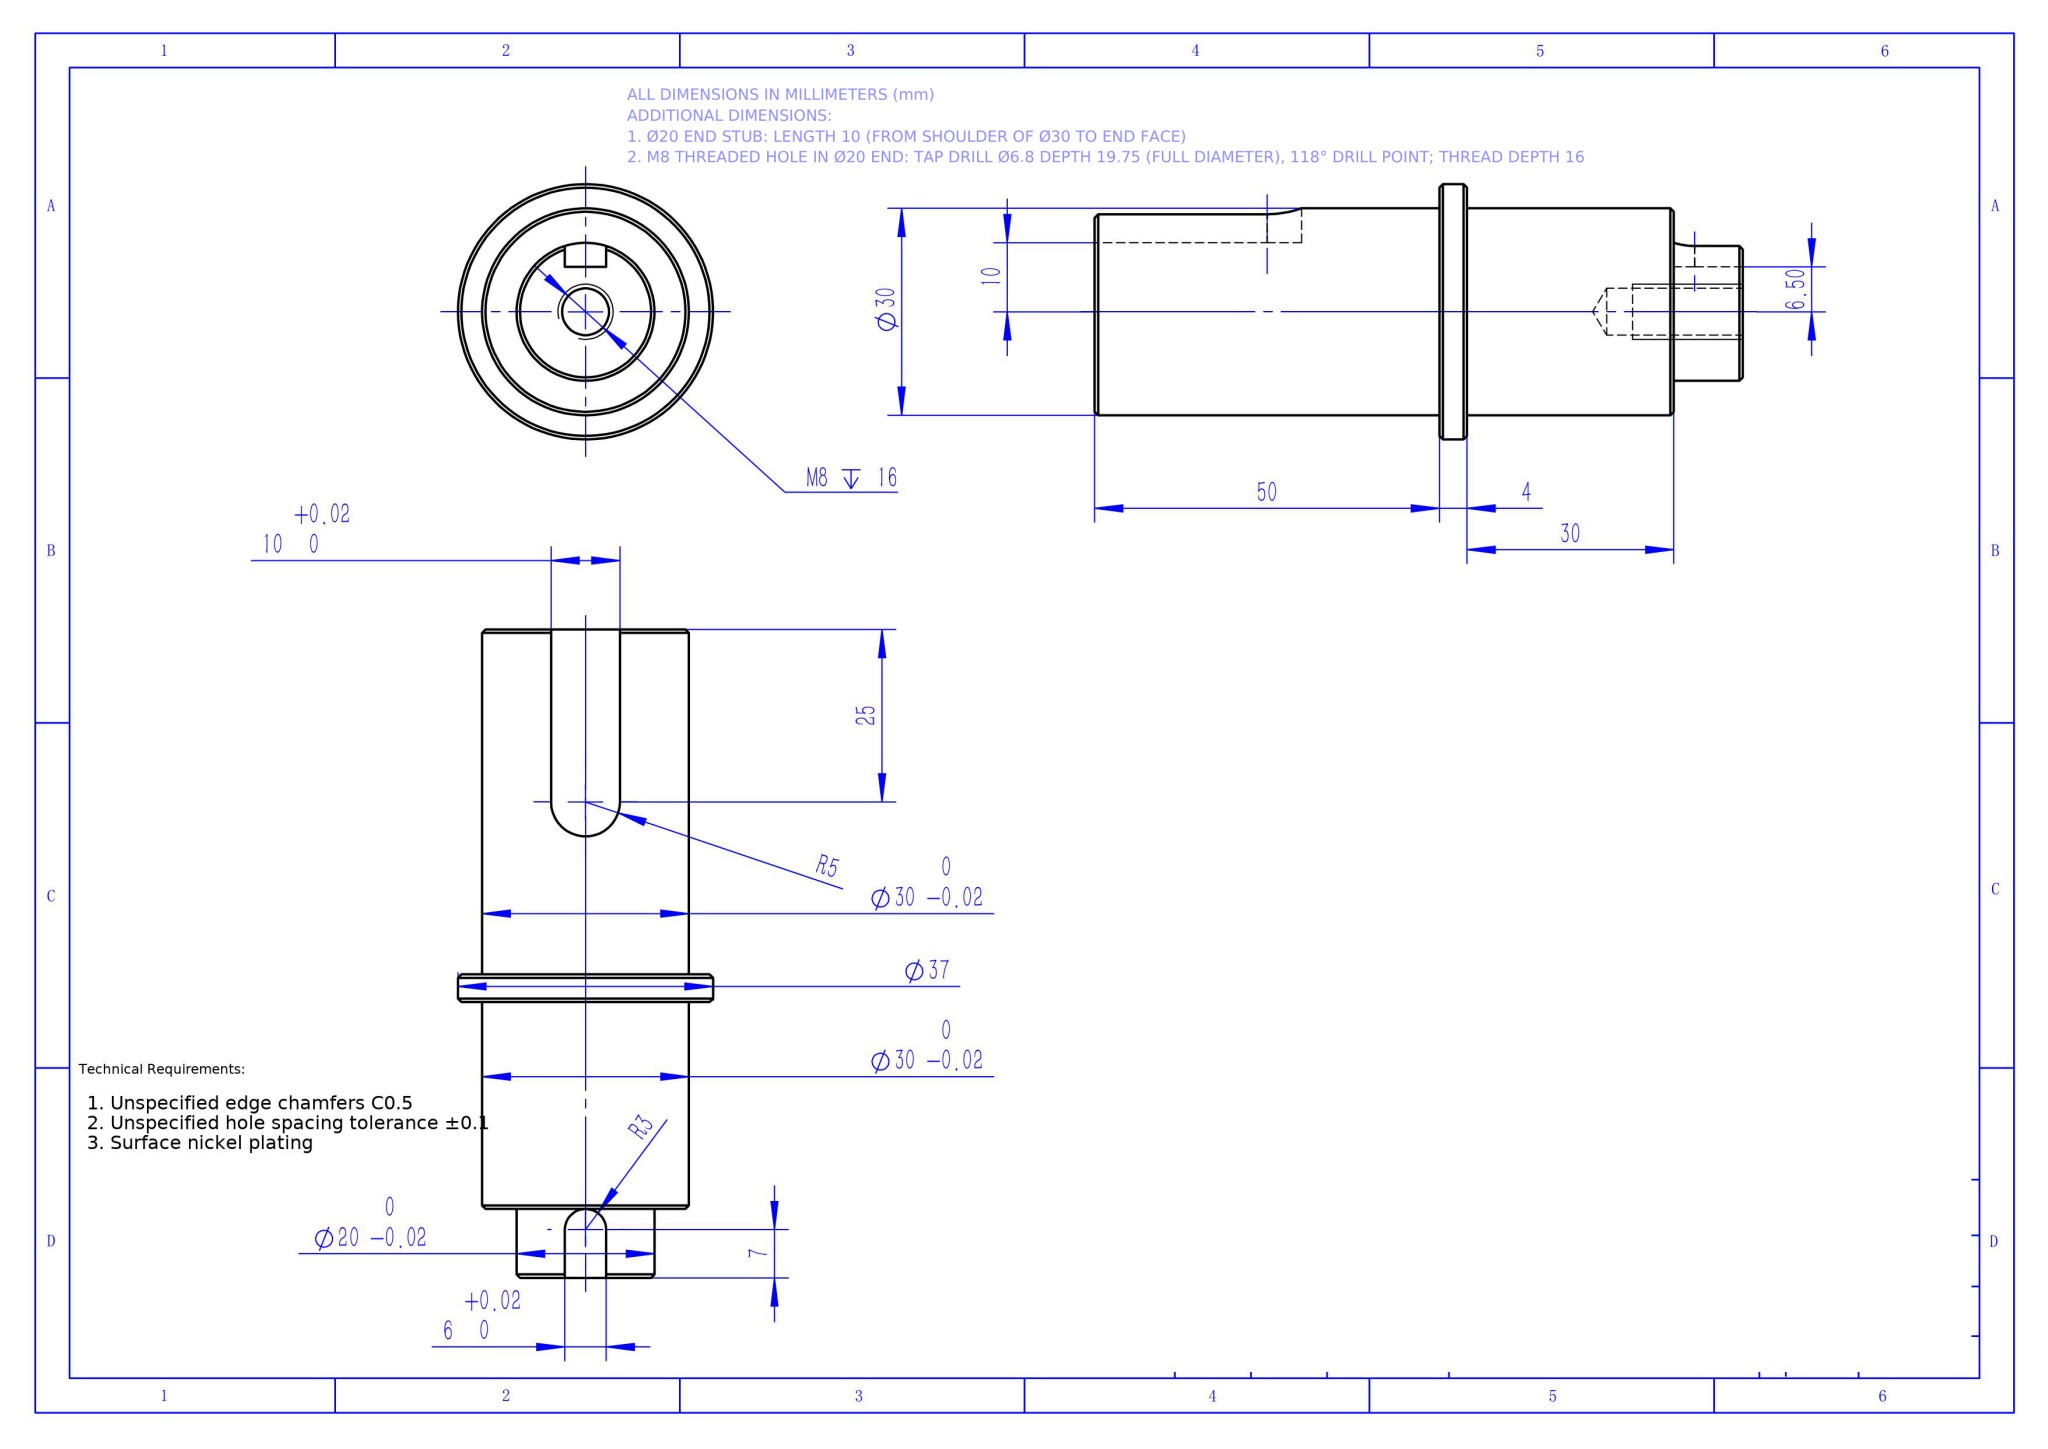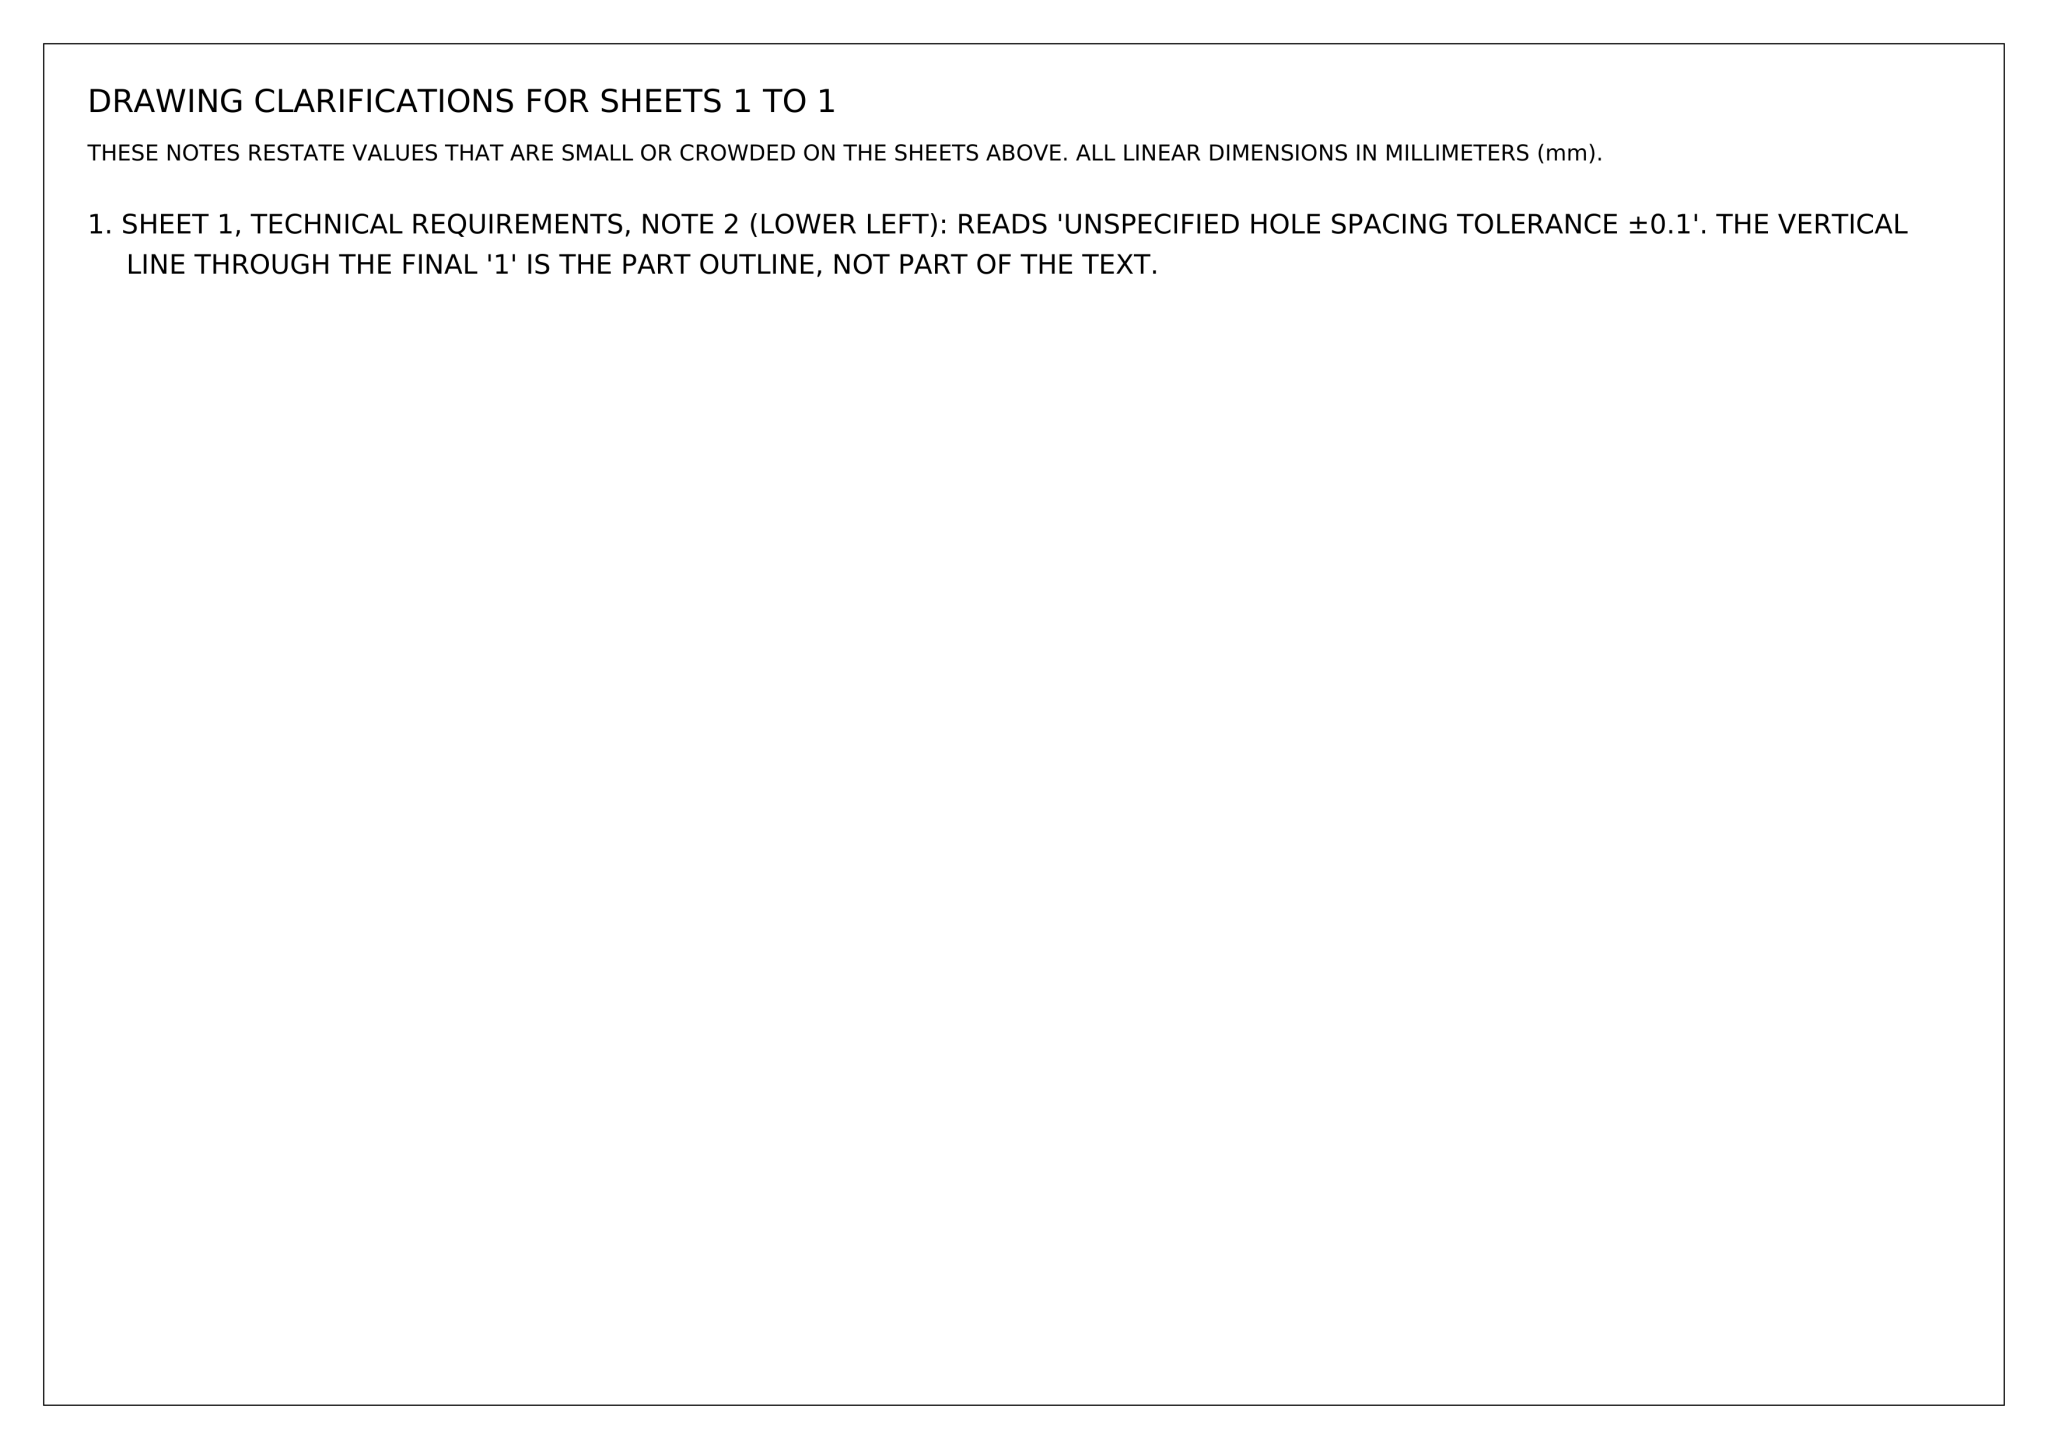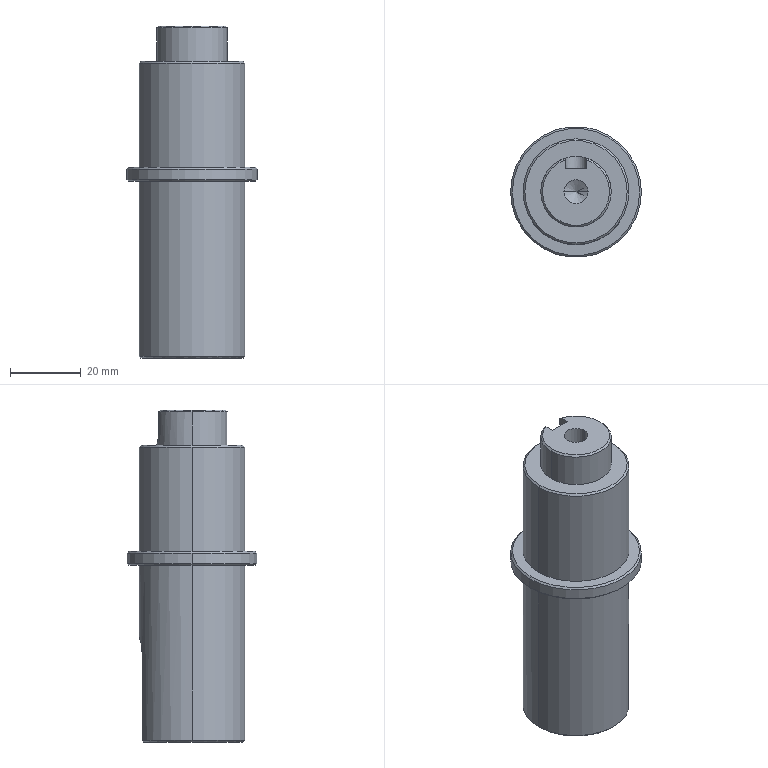Part | NX | mm | 1 solid | 39 faces | box 37 x 37 x 94 mm | volume 61635 mm3 | cone 14 | cylinder 14 | plane 11 | commonest cylinder face diameters 30 x4 20 x3 6.8 x2 10 x2 37 x2 6 x1